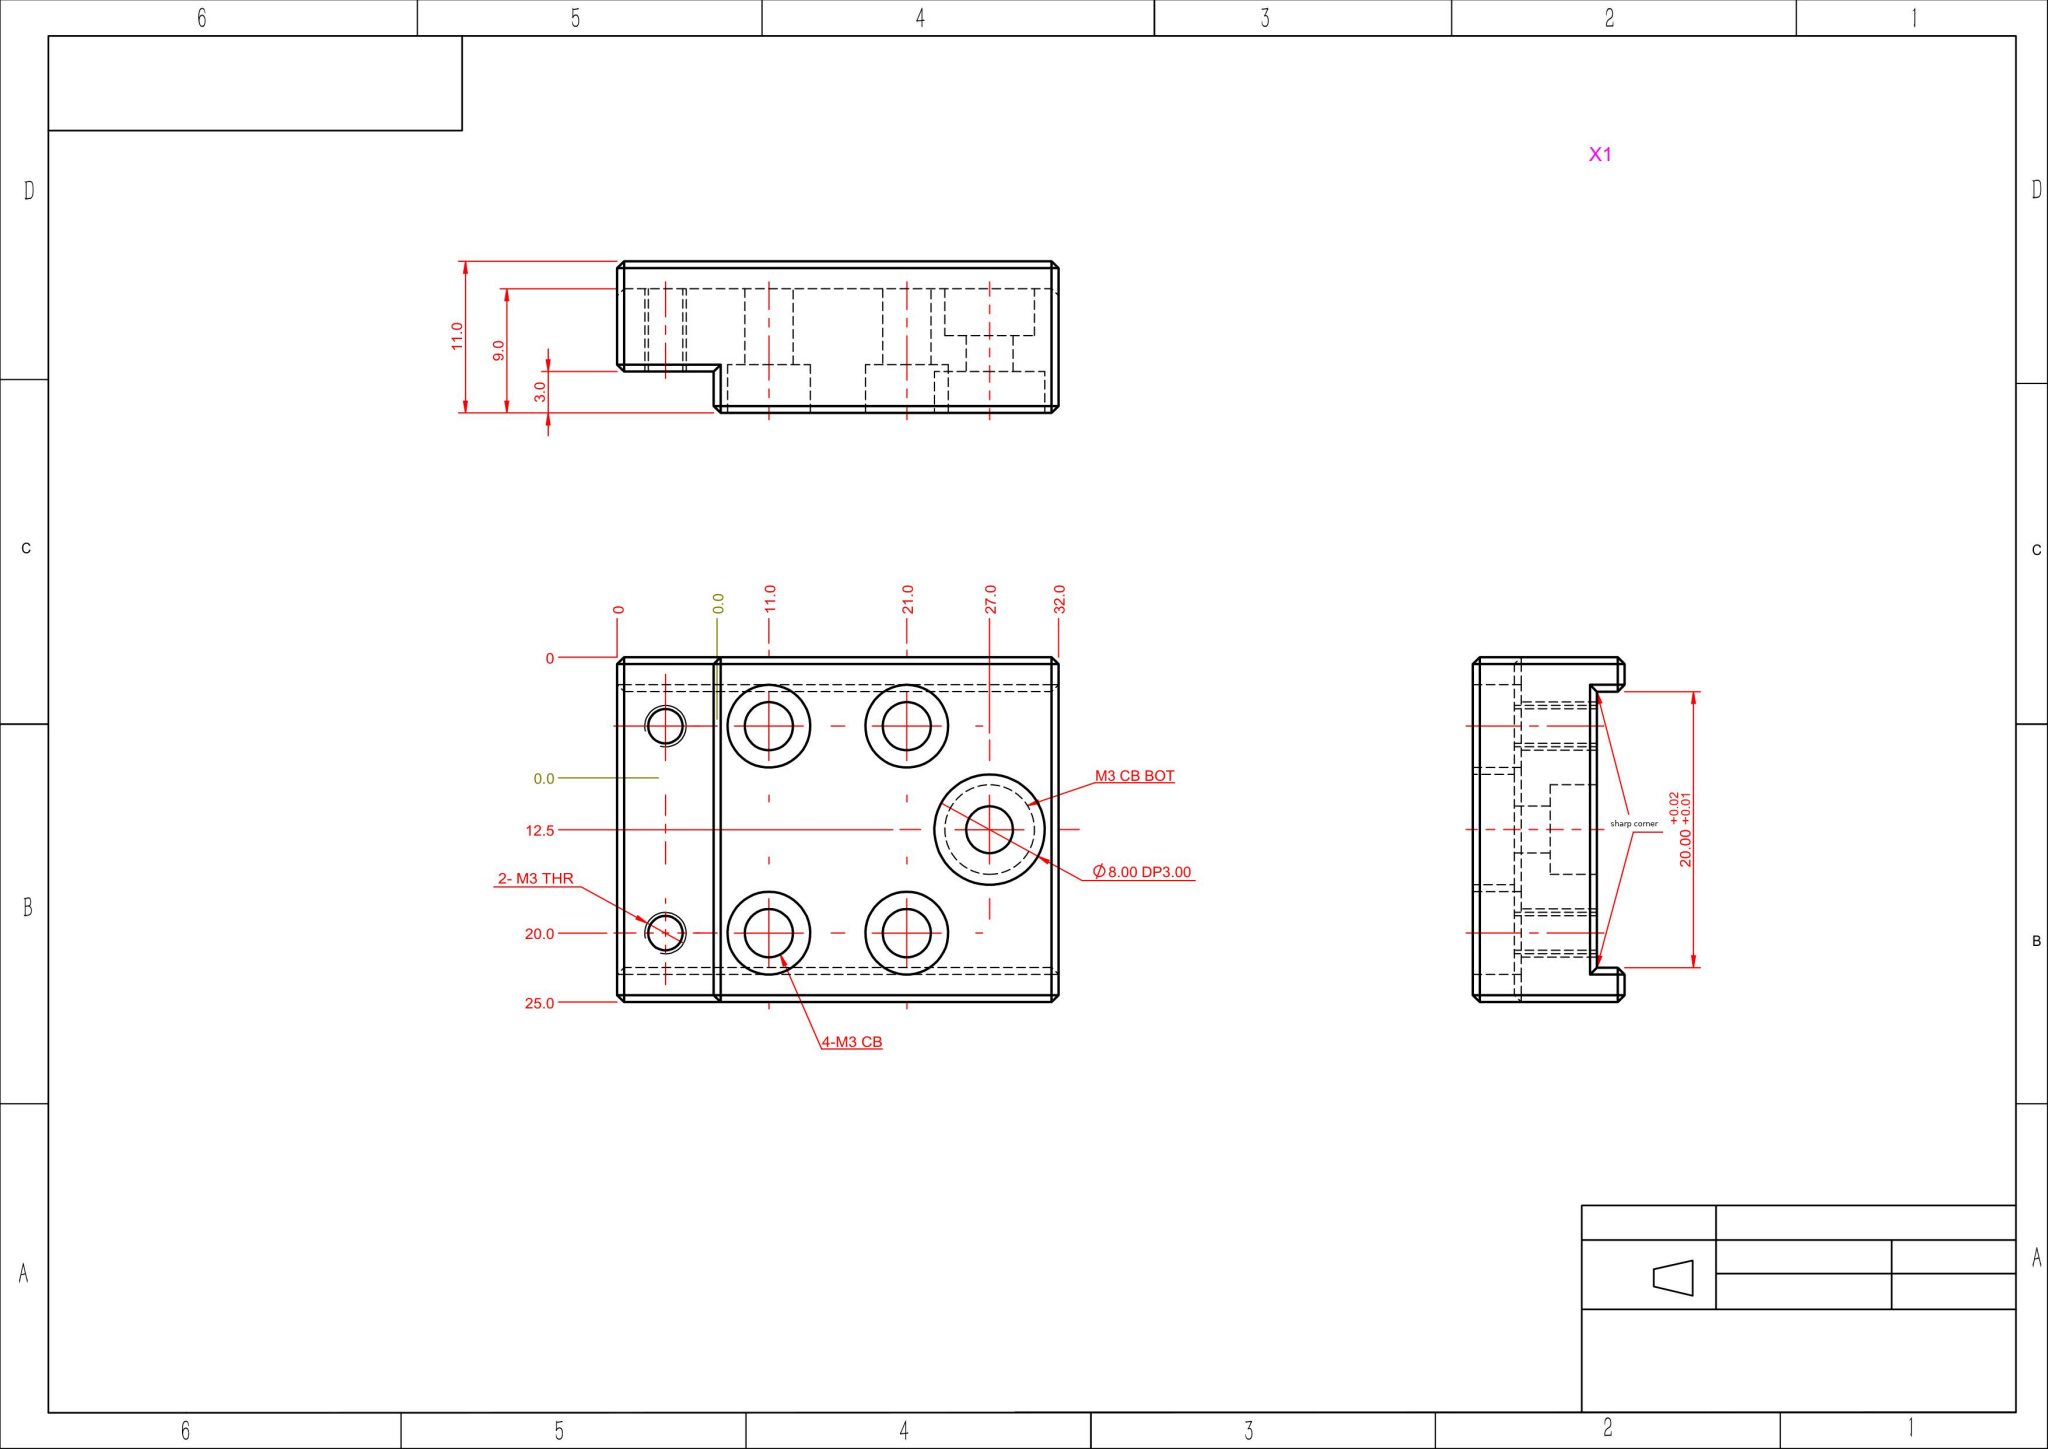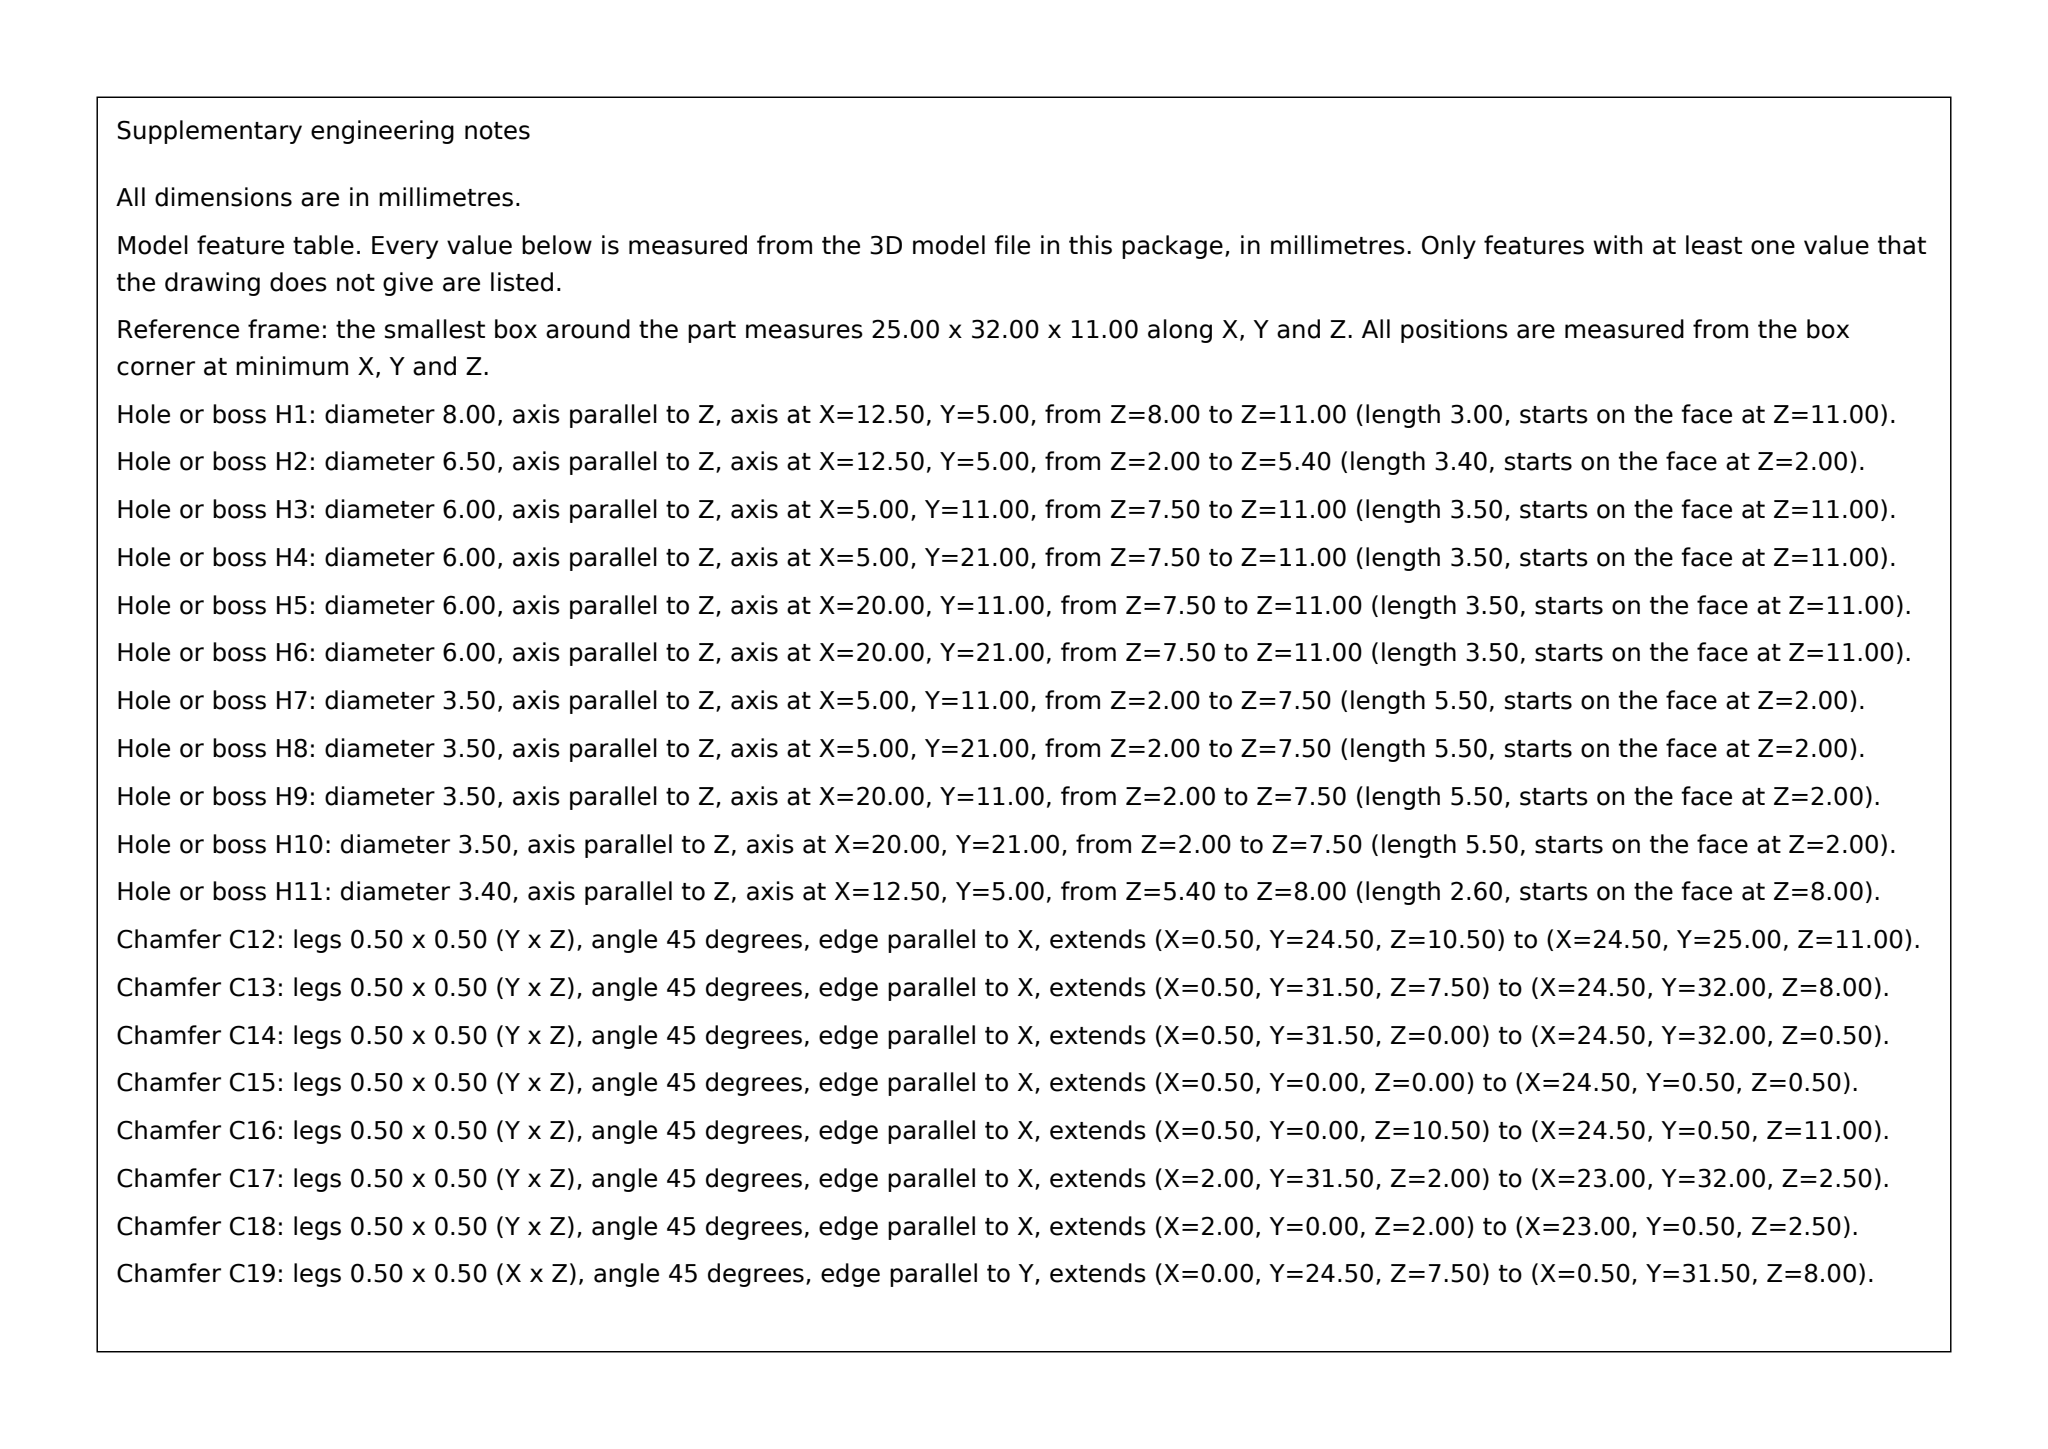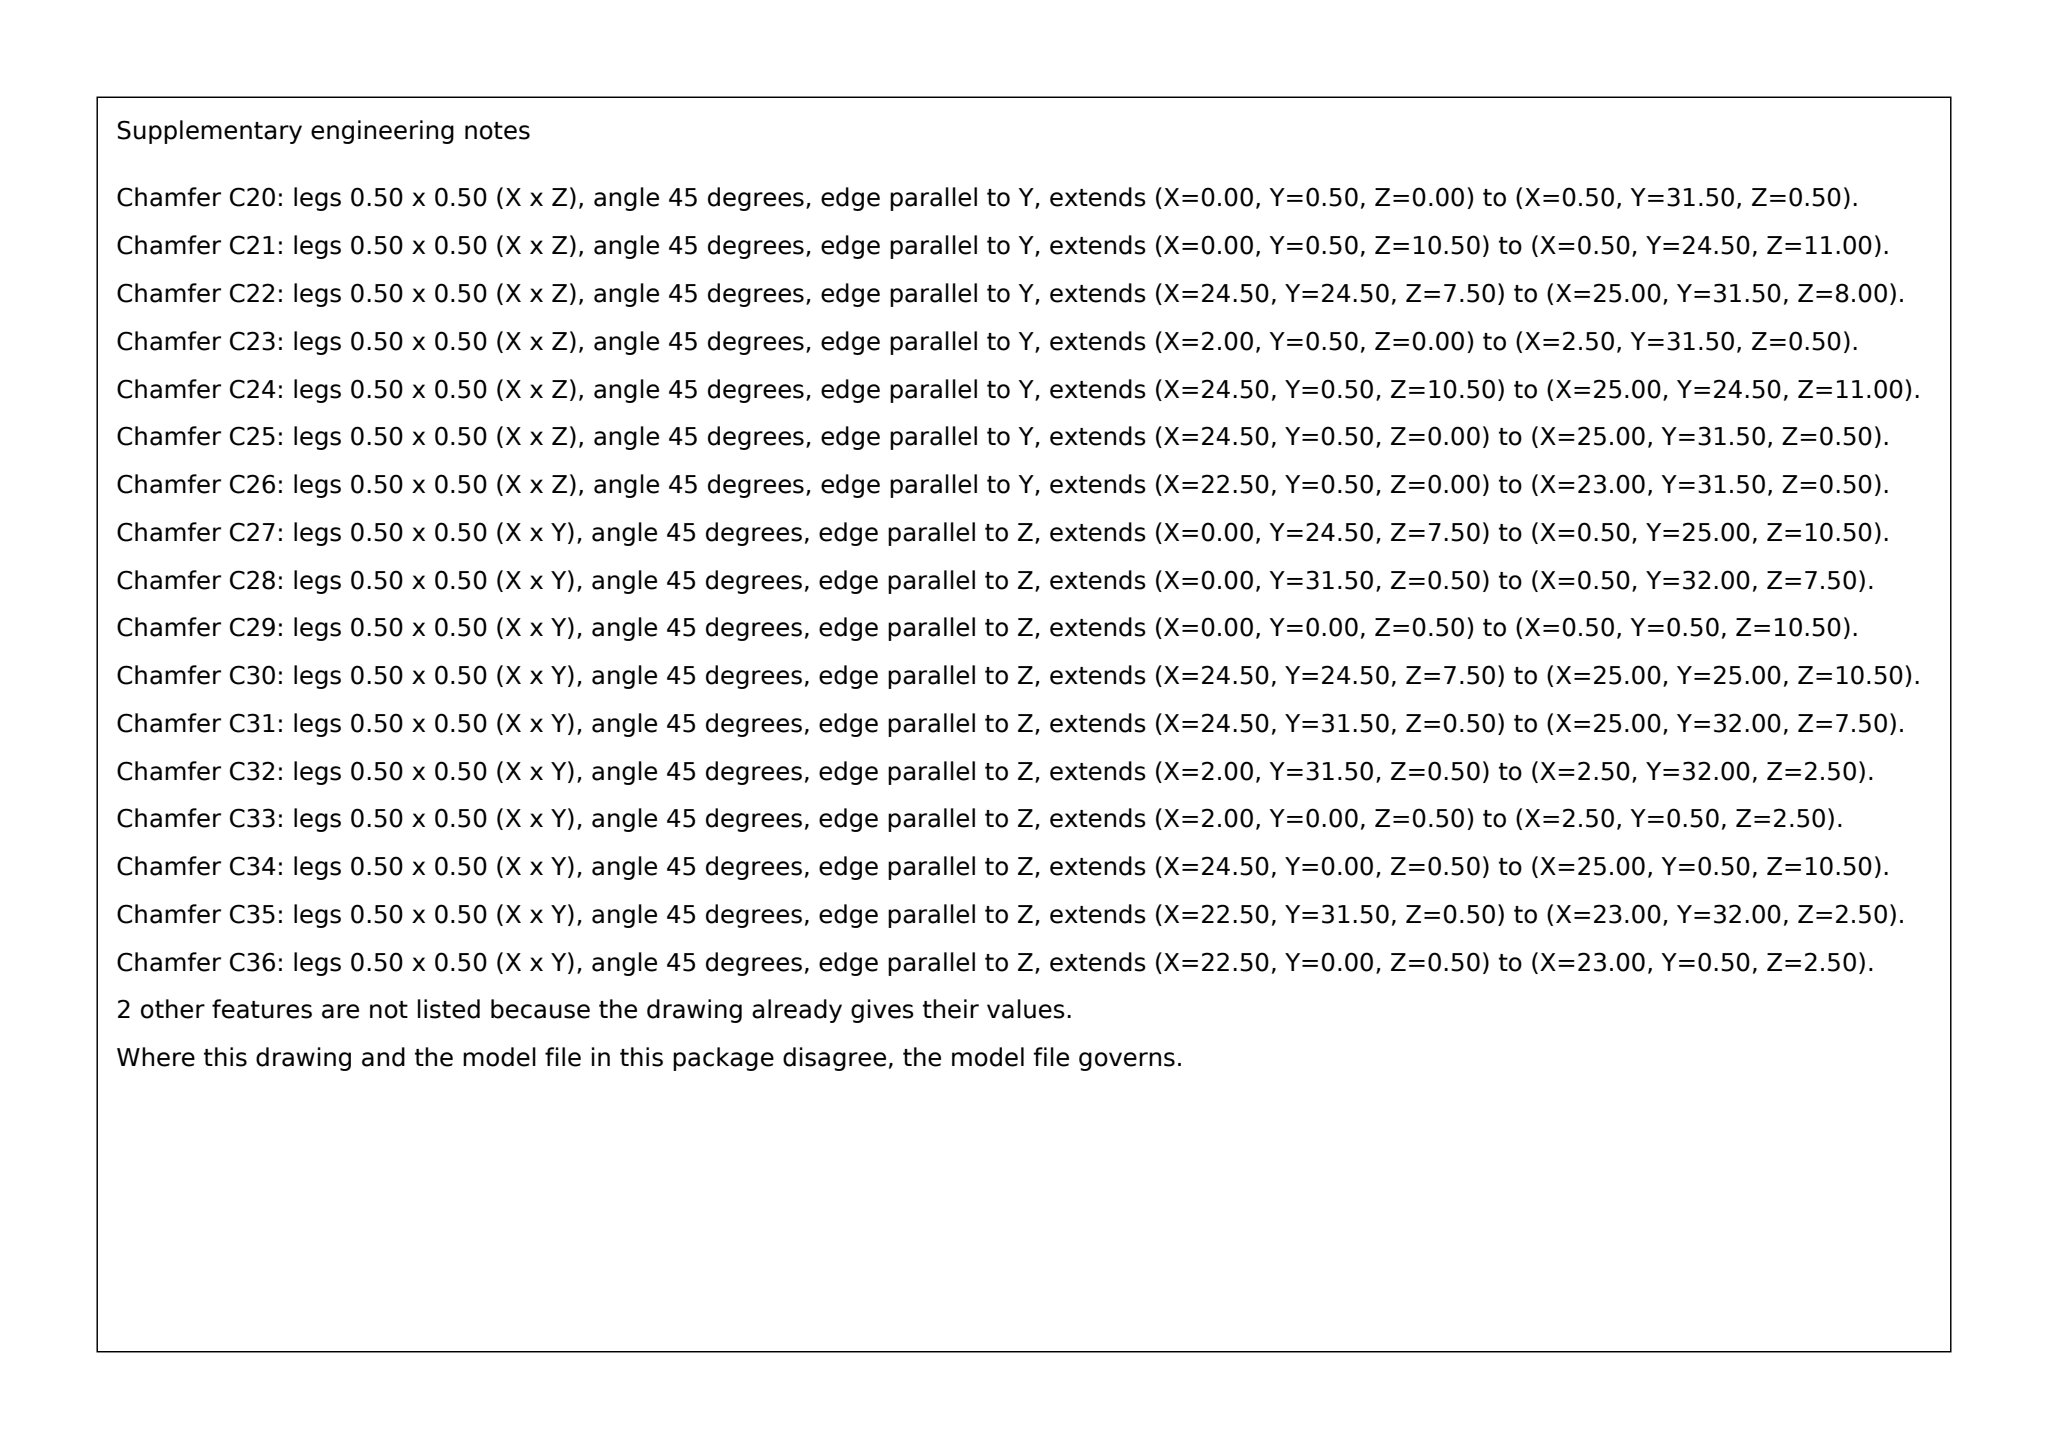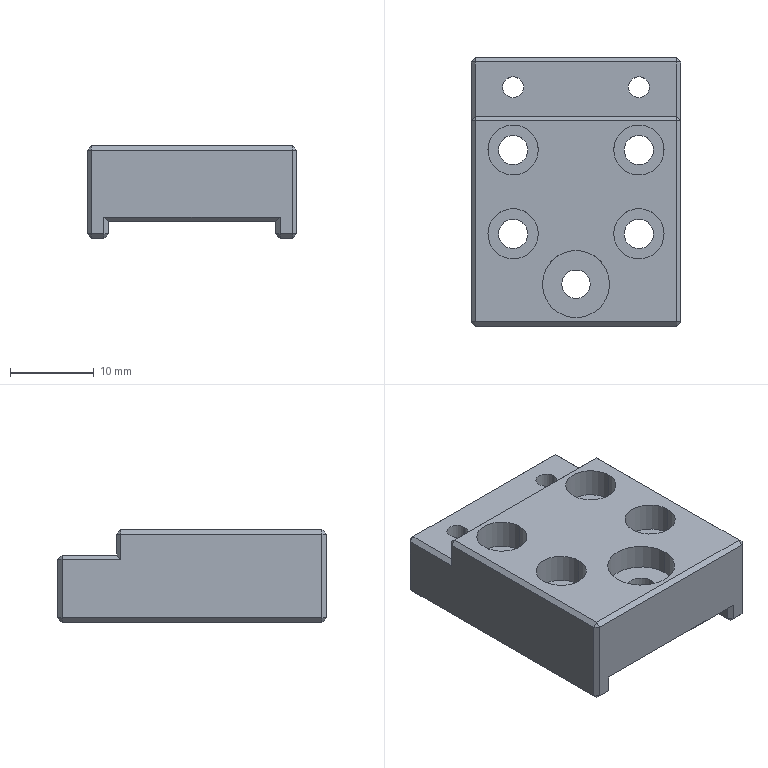Part | SolidWorks | mm | 1 solid | 85 faces | box 25 x 32 x 11 mm | volume 5996 mm3 | plane 59 | cylinder 26 | commonest cylinder face diameters 6 x8 3.5 x8 2.5 x4 6.5 x2 3.4 x2 8 x2
build123d program:
from build123d import *

# Parameters (mm, degrees)
SKETCH1_W                                            = 25
SKETCH1_H                                            = 32
BOSS_EXTRUDE1_DEPTH                                  = 11
SKETCH2_W                                            = 20
SKETCH2_H                                            = 32
CUT_EXTRUDE1_DEPTH                                   = 2
CYLINDRICAL_COUNTERSUNK_HOLE1_FOR_M3_HEX_D           = 3.5
CYLINDRICAL_COUNTERSUNK_HOLE1_FOR_M3_HEX_CBORE_D     = 6
CYLINDRICAL_COUNTERSUNK_HOLE1_FOR_M3_HEX_CBORE_DEPTH = 3.5
SKETCH5_R                                            = 4
CUT_EXTRUDE2_DEPTH                                   = 3
M3_TAPPED_HOLE1_D                                    = 2.5
LPATTERN1_COUNT                                      = 2
LPATTERN1_PITCH                                      = 15
SKETCH12_W                                           = 25
SKETCH12_H                                           = 7
CUT_EXTRUDE4_DEPTH                                   = 3
CHAMFER1_SIZE                                        = 0.5
M3_HEX_SOCKET_HEAD_CAP_SCREW_CBORE1_D                = 3.4
M3_HEX_SOCKET_HEAD_CAP_SCREW_CBORE1_CBORE_D          = 6.5
M3_HEX_SOCKET_HEAD_CAP_SCREW_CBORE1_CBORE_DEPTH      = 3.4


with BuildPart() as part:
    # Sketch1 → Boss-Extrude1 (new body)
    with BuildSketch(Plane.XY):
        Rectangle(SKETCH1_W, SKETCH1_H)
    extrude(amount=BOSS_EXTRUDE1_DEPTH)

    # Sketch2 → Cut-Extrude1 (cut)
    with BuildSketch(Plane(origin=(0, 0, 0), x_dir=(-1, 0, 0), z_dir=(0, 0, -1))):
        Rectangle(SKETCH2_W, SKETCH2_H)
    extrude(amount=-CUT_EXTRUDE1_DEPTH, mode=Mode.SUBTRACT)

    # Cylindrical Countersunk Hole1 for M3 Hex (through all)
    with Locations(Plane.XY.offset(11)):
        with Locations((-7.5, 5), (7.5, 5), (-7.5, -5), (7.5, -5)):
            CounterBoreHole(CYLINDRICAL_COUNTERSUNK_HOLE1_FOR_M3_HEX_D / 2, CYLINDRICAL_COUNTERSUNK_HOLE1_FOR_M3_HEX_CBORE_D / 2, CYLINDRICAL_COUNTERSUNK_HOLE1_FOR_M3_HEX_CBORE_DEPTH)

    # Sketch5 → Cut-Extrude2 (cut)
    with BuildSketch(Plane.XY.offset(11)):
        with Locations((0, -11)):
            Circle(SKETCH5_R)
    extrude(amount=-CUT_EXTRUDE2_DEPTH, mode=Mode.SUBTRACT)

    # M3 Tapped Hole1 (through all)
    with Locations(Plane.XY.offset(11)):
        with Locations((-7.5, 12.5)):
            m3_tapped_hole1 = Hole(M3_TAPPED_HOLE1_D / 2)

    # LPattern1: M3 Tapped Hole1 ×2
    with Locations(*[(i * LPATTERN1_PITCH, 0, 0) for i in range(1, LPATTERN1_COUNT)]):
        add(m3_tapped_hole1, mode=Mode.SUBTRACT)

    # Sketch12 → Cut-Extrude4 (cut)
    with BuildSketch(Plane.XY.offset(11)):
        with Locations((0, 12.5)):
            Rectangle(SKETCH12_W, SKETCH12_H)
    extrude(amount=-CUT_EXTRUDE4_DEPTH, mode=Mode.SUBTRACT)

    # Chamfer1
    chamfer1_edges = [part.edges().sort_by_distance(p)[0] for p in [
        (12.5, -3.5, 11),
        (-11.25, 16, 0),
        (11.25, -16, 0),
        (10, -16, 1),
        (0, 16, 2),
        (10, 16, 1),
        (-10, 16, 1),
        (0, -16, 2),
        (-10, -16, 1),
        (10, 0, 0),
        (-10, 0, 0),
        (11.25, 16, 0),
        (12.5, 0, 0),
        (-11.25, -16, 0),
        (-12.5, 0, 0),
        (0, -16, 11),
        (-12.5, -3.5, 11),
        (12.5, -16, 5.5),
        (-12.5, 16, 4),
        (12.5, 16, 4),
        (-12.5, -16, 5.5),
        (0, 9, 11),
        (-12.5, 12.5, 8),
        (-12.5, 9, 9.5),
        (0, 16, 8),
        (12.5, 12.5, 8),
        (12.5, 9, 9.5),
    ]]
    chamfer(chamfer1_edges, length=CHAMFER1_SIZE)

    # M3 Hex Socket Head Cap Screw CBORE1 (through all)
    with Locations(Plane(origin=(0, 0, 2), x_dir=(-1, 0, 0), z_dir=(0, 0, -1))):
        with Locations((0, -11)):
            CounterBoreHole(M3_HEX_SOCKET_HEAD_CAP_SCREW_CBORE1_D / 2, M3_HEX_SOCKET_HEAD_CAP_SCREW_CBORE1_CBORE_D / 2, M3_HEX_SOCKET_HEAD_CAP_SCREW_CBORE1_CBORE_DEPTH)


solid = part.part